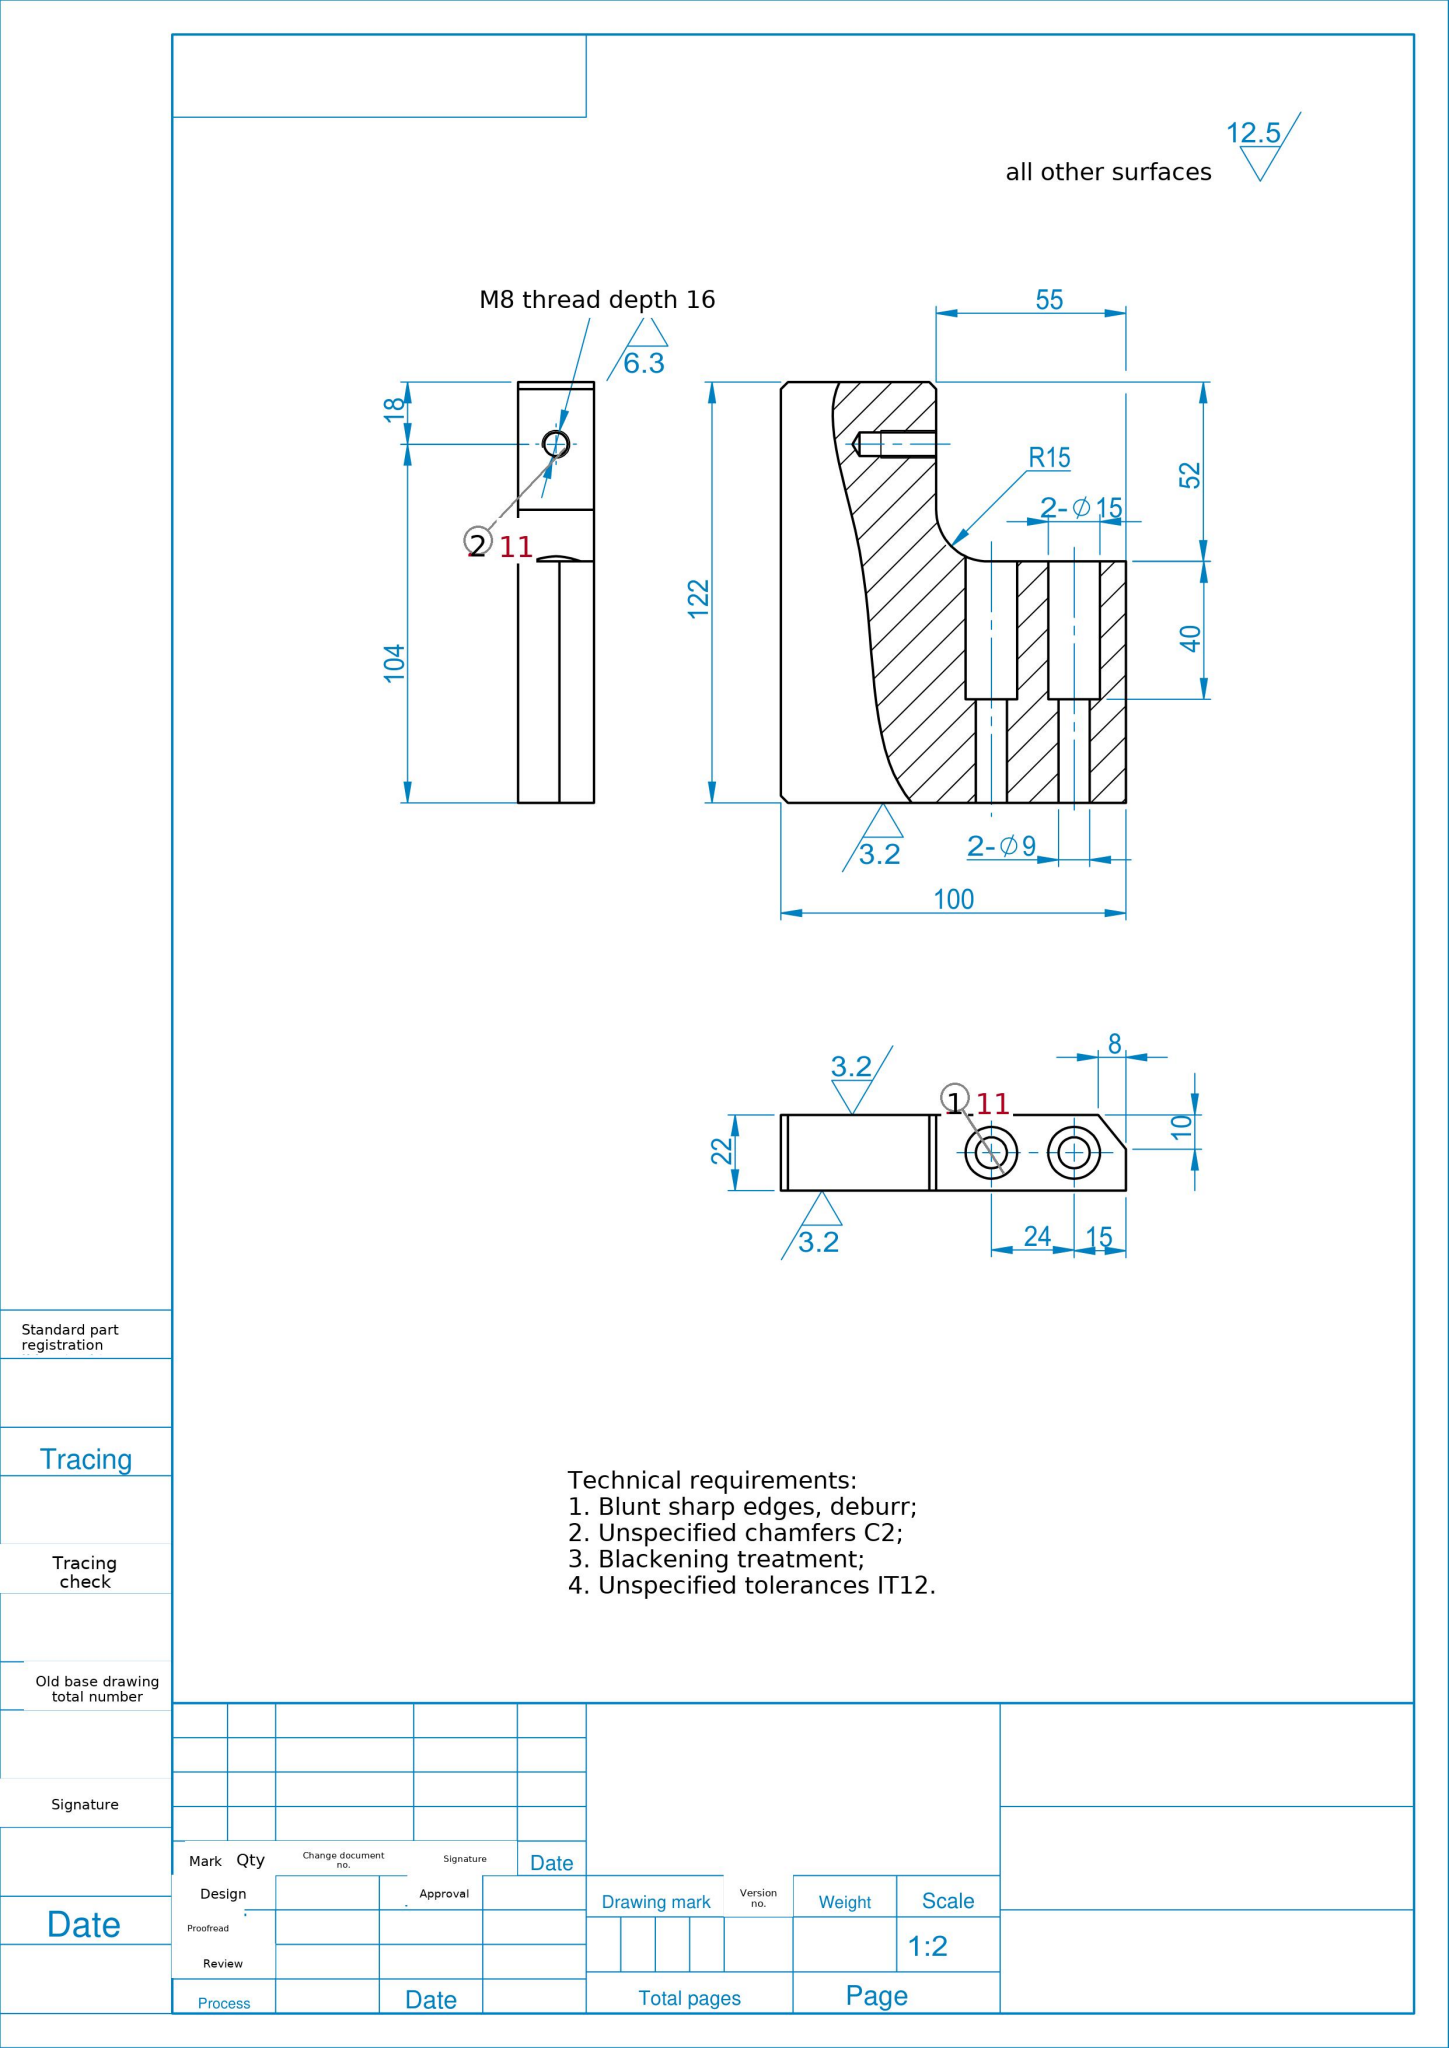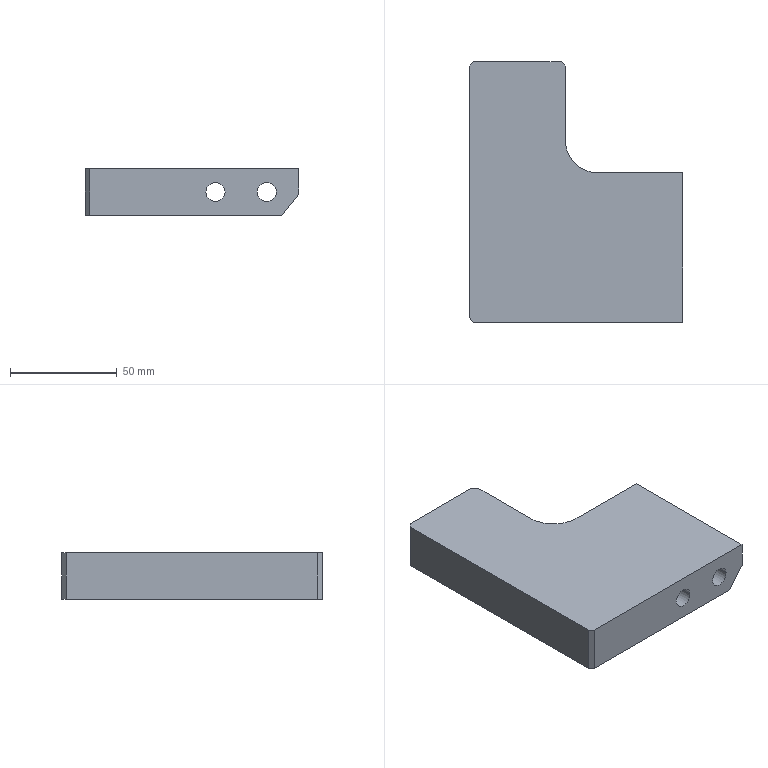Part | SolidWorks | mm | 1 solid | 27 faces | box 100 x 122 x 22 mm | volume 184797 mm3 | plane 14 | cylinder 11 | cone 2 | commonest cylinder face diameters 15 x4 9 x4 6.8 x2 30 x1
STEP:
#1=CARTESIAN_POINT('',(22.75,104.,14.4));
#2=VERTEX_POINT('',#1);
#3=CARTESIAN_POINT('',(22.75,104.,7.6));
#4=VERTEX_POINT('',#3);
#5=CARTESIAN_POINT('',(22.75,104.,11.));
#6=DIRECTION('',(1.,0.,0.));
#7=DIRECTION('',(0.,0.,-1.));
#8=AXIS2_PLACEMENT_3D('',#5,#6,#7);
#9=CIRCLE('',#8,3.4);
#10=EDGE_CURVE('',#2,#4,#9,.T.);
#11=ORIENTED_EDGE('',*,*,#10,.F.);
#12=CARTESIAN_POINT('',(45.,104.,14.4));
#13=VERTEX_POINT('',#12);
#14=CARTESIAN_POINT('',(45.,104.,14.4));
#15=DIRECTION('',(1.,0.,0.));
#16=VECTOR('',#15,1000.);
#17=LINE('',#14,#16);
#18=EDGE_CURVE('',#2,#13,#17,.T.);
#19=ORIENTED_EDGE('',*,*,#18,.T.);
#20=CARTESIAN_POINT('',(45.,104.,7.6));
#21=VERTEX_POINT('',#20);
#22=CARTESIAN_POINT('',(45.,104.,11.));
#23=DIRECTION('',(1.,0.,0.));
#24=DIRECTION('',(0.,0.,-1.));
#25=AXIS2_PLACEMENT_3D('',#22,#23,#24);
#26=CIRCLE('',#25,3.4);
#27=EDGE_CURVE('',#13,#21,#26,.T.);
#28=ORIENTED_EDGE('',*,*,#27,.T.);
#29=CARTESIAN_POINT('',(45.,104.,7.6));
#30=DIRECTION('',(1.,0.,0.));
#31=VECTOR('',#30,1000.);
#32=LINE('',#29,#31);
#33=EDGE_CURVE('',#4,#21,#32,.T.);
#34=ORIENTED_EDGE('',*,*,#33,.F.);
#35=EDGE_LOOP('',(#11,#19,#28,#34));
#36=FACE_OUTER_BOUND('',#35,.T.);
#37=CARTESIAN_POINT('',(45.,104.,11.));
#38=DIRECTION('',(1.,0.,0.));
#39=DIRECTION('',(0.,0.,-1.));
#40=AXIS2_PLACEMENT_3D('',#37,#38,#39);
#41=CYLINDRICAL_SURFACE('',#40,3.4);
#42=ADVANCED_FACE('',(#36),#41,.F.);
#43=CARTESIAN_POINT('',(20.707,104.,11.));
#44=VERTEX_POINT('',#43);
#45=CARTESIAN_POINT('',(22.75,104.,7.6));
#46=DIRECTION('',(0.515,0.,-0.8572));
#47=VECTOR('',#46,1000.);
#48=LINE('',#45,#47);
#49=EDGE_CURVE('',#44,#4,#48,.T.);
#50=ORIENTED_EDGE('',*,*,#49,.F.);
#51=CARTESIAN_POINT('',(22.75,104.,14.4));
#52=DIRECTION('',(0.515,0.,0.8572));
#53=VECTOR('',#52,1000.);
#54=LINE('',#51,#53);
#55=EDGE_CURVE('',#44,#2,#54,.T.);
#56=ORIENTED_EDGE('',*,*,#55,.T.);
#57=ORIENTED_EDGE('',*,*,#10,.T.);
#58=EDGE_LOOP('',(#50,#56,#57));
#59=FACE_OUTER_BOUND('',#58,.T.);
#60=CARTESIAN_POINT('',(22.75,104.,11.));
#61=DIRECTION('',(1.,0.,0.));
#62=DIRECTION('',(0.,0.,-1.));
#63=AXIS2_PLACEMENT_3D('',#60,#61,#62);
#64=CONICAL_SURFACE('',#63,3.4,1.03);
#65=ADVANCED_FACE('',(#59),#64,.F.);
#66=CARTESIAN_POINT('',(92.5,30.,11.));
#67=VERTEX_POINT('',#66);
#68=CARTESIAN_POINT('',(77.5,30.,11.));
#69=VERTEX_POINT('',#68);
#70=CARTESIAN_POINT('',(85.,30.,11.));
#71=DIRECTION('',(-0.,1.,0.));
#72=DIRECTION('',(-1.,-0.,0.));
#73=AXIS2_PLACEMENT_3D('',#70,#71,#72);
#74=CIRCLE('',#73,7.5);
#75=EDGE_CURVE('',#67,#69,#74,.T.);
#76=ORIENTED_EDGE('',*,*,#75,.F.);
#77=CARTESIAN_POINT('',(92.5,70.,11.));
#78=VERTEX_POINT('',#77);
#79=CARTESIAN_POINT('',(92.5,30.,11.));
#80=DIRECTION('',(-0.,1.,0.));
#81=VECTOR('',#80,1000.);
#82=LINE('',#79,#81);
#83=EDGE_CURVE('',#67,#78,#82,.T.);
#84=ORIENTED_EDGE('',*,*,#83,.T.);
#85=CARTESIAN_POINT('',(77.5,70.,11.));
#86=VERTEX_POINT('',#85);
#87=CARTESIAN_POINT('',(85.,70.,11.));
#88=DIRECTION('',(0.,-1.,0.));
#89=DIRECTION('',(1.,0.,0.));
#90=AXIS2_PLACEMENT_3D('',#87,#88,#89);
#91=CIRCLE('',#90,7.5);
#92=EDGE_CURVE('',#86,#78,#91,.T.);
#93=ORIENTED_EDGE('',*,*,#92,.F.);
#94=CARTESIAN_POINT('',(77.5,30.,11.));
#95=DIRECTION('',(-0.,1.,0.));
#96=VECTOR('',#95,1000.);
#97=LINE('',#94,#96);
#98=EDGE_CURVE('',#69,#86,#97,.T.);
#99=ORIENTED_EDGE('',*,*,#98,.F.);
#100=EDGE_LOOP('',(#76,#84,#93,#99));
#101=FACE_OUTER_BOUND('',#100,.T.);
#102=CARTESIAN_POINT('',(85.,30.,11.));
#103=DIRECTION('',(-0.,1.,0.));
#104=DIRECTION('',(-1.,-0.,0.));
#105=AXIS2_PLACEMENT_3D('',#102,#103,#104);
#106=CYLINDRICAL_SURFACE('',#105,7.5);
#107=ADVANCED_FACE('',(#101),#106,.F.);
#108=CARTESIAN_POINT('',(68.5,30.,11.));
#109=VERTEX_POINT('',#108);
#110=CARTESIAN_POINT('',(53.5,30.,11.));
#111=VERTEX_POINT('',#110);
#112=CARTESIAN_POINT('',(61.,30.,11.));
#113=DIRECTION('',(-0.,1.,0.));
#114=DIRECTION('',(-1.,-0.,0.));
#115=AXIS2_PLACEMENT_3D('',#112,#113,#114);
#116=CIRCLE('',#115,7.5);
#117=EDGE_CURVE('',#109,#111,#116,.T.);
#118=ORIENTED_EDGE('',*,*,#117,.F.);
#119=CARTESIAN_POINT('',(68.5,70.,11.));
#120=VERTEX_POINT('',#119);
#121=CARTESIAN_POINT('',(68.5,30.,11.));
#122=DIRECTION('',(-0.,1.,0.));
#123=VECTOR('',#122,1000.);
#124=LINE('',#121,#123);
#125=EDGE_CURVE('',#109,#120,#124,.T.);
#126=ORIENTED_EDGE('',*,*,#125,.T.);
#127=CARTESIAN_POINT('',(60.,70.,3.567));
#128=VERTEX_POINT('',#127);
#129=CARTESIAN_POINT('',(61.,70.,11.));
#130=DIRECTION('',(0.,-1.,0.));
#131=DIRECTION('',(1.,0.,0.));
#132=AXIS2_PLACEMENT_3D('',#129,#130,#131);
#133=CIRCLE('',#132,7.5);
#134=EDGE_CURVE('',#128,#120,#133,.T.);
#135=ORIENTED_EDGE('',*,*,#134,.F.);
#136=CARTESIAN_POINT('',(53.5,71.481,11.));
#137=VERTEX_POINT('',#136);
#138=CARTESIAN_POINT('',(53.5,71.481,11.));
#139=CARTESIAN_POINT('',(53.5,71.481,10.541));
#140=CARTESIAN_POINT('',(53.542,71.461,10.09));
#141=CARTESIAN_POINT('',(53.664,71.404,9.426));
#142=CARTESIAN_POINT('',(53.714,71.38,9.206));
#143=CARTESIAN_POINT('',(53.835,71.325,8.771));
#144=CARTESIAN_POINT('',(53.906,71.293,8.554));
#145=CARTESIAN_POINT('',(54.146,71.188,7.922));
#146=CARTESIAN_POINT('',(54.341,71.106,7.522));
#147=CARTESIAN_POINT('',(54.799,70.929,6.759));
#148=CARTESIAN_POINT('',(55.064,70.832,6.394));
#149=CARTESIAN_POINT('',(55.649,70.642,5.726));
#150=CARTESIAN_POINT('',(55.968,70.547,5.42));
#151=CARTESIAN_POINT('',(56.665,70.371,4.864));
#152=CARTESIAN_POINT('',(57.043,70.289,4.613));
#153=CARTESIAN_POINT('',(57.83,70.152,4.188));
#154=CARTESIAN_POINT('',(58.241,70.097,4.011));
#155=CARTESIAN_POINT('',(58.887,70.04,3.8));
#156=CARTESIAN_POINT('',(59.108,70.025,3.739));
#157=CARTESIAN_POINT('',(59.553,70.005,3.637));
#158=CARTESIAN_POINT('',(59.776,70.,3.597));
#159=CARTESIAN_POINT('',(60.,70.,3.567));
#160=B_SPLINE_CURVE_WITH_KNOTS('',3,(#138,#139,#140,#141,#142,#143,#144,#145,#146,#147,#148,#149,#150,#151,#152,#153,#154,#155,#156,#157,#158,#159),.UNSPECIFIED.,.F.,.F.,(4,2,2,2,2,2,2,2,2,2,4),(0.,0.001356,0.002034,0.002712,0.004067,0.005423,0.006779,0.008135,0.009491,0.01017,0.01085),.UNSPECIFIED.);
#161=EDGE_CURVE('',#137,#128,#160,.T.);
#162=ORIENTED_EDGE('',*,*,#161,.F.);
#163=CARTESIAN_POINT('',(53.5,30.,11.));
#164=DIRECTION('',(-0.,1.,0.));
#165=VECTOR('',#164,1000.);
#166=LINE('',#163,#165);
#167=EDGE_CURVE('',#111,#137,#166,.T.);
#168=ORIENTED_EDGE('',*,*,#167,.F.);
#169=EDGE_LOOP('',(#118,#126,#135,#162,#168));
#170=FACE_OUTER_BOUND('',#169,.T.);
#171=CARTESIAN_POINT('',(61.,30.,11.));
#172=DIRECTION('',(-0.,1.,0.));
#173=DIRECTION('',(-1.,-0.,0.));
#174=AXIS2_PLACEMENT_3D('',#171,#172,#173);
#175=CYLINDRICAL_SURFACE('',#174,7.5);
#176=ADVANCED_FACE('',(#170),#175,.F.);
#177=CARTESIAN_POINT('',(65.5,30.,11.));
#178=VERTEX_POINT('',#177);
#179=CARTESIAN_POINT('',(56.5,30.,11.));
#180=VERTEX_POINT('',#179);
#181=CARTESIAN_POINT('',(61.,30.,11.));
#182=DIRECTION('',(-0.,1.,0.));
#183=DIRECTION('',(-1.,0.,0.));
#184=AXIS2_PLACEMENT_3D('',#181,#182,#183);
#185=CIRCLE('',#184,4.5);
#186=EDGE_CURVE('',#178,#180,#185,.T.);
#187=ORIENTED_EDGE('',*,*,#186,.T.);
#188=CARTESIAN_POINT('',(56.5,-0.,11.));
#189=VERTEX_POINT('',#188);
#190=CARTESIAN_POINT('',(56.5,80.,11.));
#191=DIRECTION('',(0.,-1.,0.));
#192=VECTOR('',#191,1000.);
#193=LINE('',#190,#192);
#194=EDGE_CURVE('',#180,#189,#193,.T.);
#195=ORIENTED_EDGE('',*,*,#194,.T.);
#196=CARTESIAN_POINT('',(65.5,-0.,11.));
#197=VERTEX_POINT('',#196);
#198=CARTESIAN_POINT('',(61.,-0.,11.));
#199=DIRECTION('',(-0.,1.,0.));
#200=DIRECTION('',(-1.,-0.,0.));
#201=AXIS2_PLACEMENT_3D('',#198,#199,#200);
#202=CIRCLE('',#201,4.5);
#203=EDGE_CURVE('',#197,#189,#202,.T.);
#204=ORIENTED_EDGE('',*,*,#203,.F.);
#205=CARTESIAN_POINT('',(65.5,80.,11.));
#206=DIRECTION('',(0.,-1.,0.));
#207=VECTOR('',#206,1000.);
#208=LINE('',#205,#207);
#209=EDGE_CURVE('',#178,#197,#208,.T.);
#210=ORIENTED_EDGE('',*,*,#209,.F.);
#211=EDGE_LOOP('',(#187,#195,#204,#210));
#212=FACE_OUTER_BOUND('',#211,.T.);
#213=CARTESIAN_POINT('',(61.,80.,11.));
#214=DIRECTION('',(0.,-1.,0.));
#215=DIRECTION('',(1.,0.,0.));
#216=AXIS2_PLACEMENT_3D('',#213,#214,#215);
#217=CYLINDRICAL_SURFACE('',#216,4.5);
#218=ADVANCED_FACE('',(#212),#217,.F.);
#219=CARTESIAN_POINT('',(89.5,30.,11.));
#220=VERTEX_POINT('',#219);
#221=CARTESIAN_POINT('',(80.5,30.,11.));
#222=VERTEX_POINT('',#221);
#223=CARTESIAN_POINT('',(85.,30.,11.));
#224=DIRECTION('',(-0.,1.,0.));
#225=DIRECTION('',(-1.,0.,0.));
#226=AXIS2_PLACEMENT_3D('',#223,#224,#225);
#227=CIRCLE('',#226,4.5);
#228=EDGE_CURVE('',#220,#222,#227,.T.);
#229=ORIENTED_EDGE('',*,*,#228,.T.);
#230=CARTESIAN_POINT('',(80.5,-0.,11.));
#231=VERTEX_POINT('',#230);
#232=CARTESIAN_POINT('',(80.5,80.,11.));
#233=DIRECTION('',(0.,-1.,0.));
#234=VECTOR('',#233,1000.);
#235=LINE('',#232,#234);
#236=EDGE_CURVE('',#222,#231,#235,.T.);
#237=ORIENTED_EDGE('',*,*,#236,.T.);
#238=CARTESIAN_POINT('',(89.5,0.,11.));
#239=VERTEX_POINT('',#238);
#240=CARTESIAN_POINT('',(85.,0.,11.));
#241=DIRECTION('',(-0.,1.,0.));
#242=DIRECTION('',(-1.,-0.,0.));
#243=AXIS2_PLACEMENT_3D('',#240,#241,#242);
#244=CIRCLE('',#243,4.5);
#245=EDGE_CURVE('',#239,#231,#244,.T.);
#246=ORIENTED_EDGE('',*,*,#245,.F.);
#247=CARTESIAN_POINT('',(89.5,80.,11.));
#248=DIRECTION('',(0.,-1.,0.));
#249=VECTOR('',#248,1000.);
#250=LINE('',#247,#249);
#251=EDGE_CURVE('',#220,#239,#250,.T.);
#252=ORIENTED_EDGE('',*,*,#251,.F.);
#253=EDGE_LOOP('',(#229,#237,#246,#252));
#254=FACE_OUTER_BOUND('',#253,.T.);
#255=CARTESIAN_POINT('',(85.,80.,11.));
#256=DIRECTION('',(0.,-1.,0.));
#257=DIRECTION('',(1.,0.,0.));
#258=AXIS2_PLACEMENT_3D('',#255,#256,#257);
#259=CYLINDRICAL_SURFACE('',#258,4.5);
#260=ADVANCED_FACE('',(#254),#259,.F.);
#261=ORIENTED_EDGE('',*,*,#236,.F.);
#262=CARTESIAN_POINT('',(85.,30.,11.));
#263=DIRECTION('',(-0.,1.,0.));
#264=DIRECTION('',(-1.,0.,0.));
#265=AXIS2_PLACEMENT_3D('',#262,#263,#264);
#266=CIRCLE('',#265,4.5);
#267=EDGE_CURVE('',#222,#220,#266,.T.);
#268=ORIENTED_EDGE('',*,*,#267,.T.);
#269=ORIENTED_EDGE('',*,*,#251,.T.);
#270=CARTESIAN_POINT('',(85.,0.,11.));
#271=DIRECTION('',(-0.,1.,0.));
#272=DIRECTION('',(-1.,-0.,0.));
#273=AXIS2_PLACEMENT_3D('',#270,#271,#272);
#274=CIRCLE('',#273,4.5);
#275=EDGE_CURVE('',#231,#239,#274,.T.);
#276=ORIENTED_EDGE('',*,*,#275,.F.);
#277=EDGE_LOOP('',(#261,#268,#269,#276));
#278=FACE_OUTER_BOUND('',#277,.T.);
#279=CARTESIAN_POINT('',(85.,80.,11.));
#280=DIRECTION('',(0.,-1.,0.));
#281=DIRECTION('',(1.,0.,0.));
#282=AXIS2_PLACEMENT_3D('',#279,#280,#281);
#283=CYLINDRICAL_SURFACE('',#282,4.5);
#284=ADVANCED_FACE('',(#278),#283,.F.);
#285=ORIENTED_EDGE('',*,*,#194,.F.);
#286=CARTESIAN_POINT('',(61.,30.,11.));
#287=DIRECTION('',(-0.,1.,0.));
#288=DIRECTION('',(-1.,0.,0.));
#289=AXIS2_PLACEMENT_3D('',#286,#287,#288);
#290=CIRCLE('',#289,4.5);
#291=EDGE_CURVE('',#180,#178,#290,.T.);
#292=ORIENTED_EDGE('',*,*,#291,.T.);
#293=ORIENTED_EDGE('',*,*,#209,.T.);
#294=CARTESIAN_POINT('',(61.,-0.,11.));
#295=DIRECTION('',(-0.,1.,0.));
#296=DIRECTION('',(-1.,-0.,0.));
#297=AXIS2_PLACEMENT_3D('',#294,#295,#296);
#298=CIRCLE('',#297,4.5);
#299=EDGE_CURVE('',#189,#197,#298,.T.);
#300=ORIENTED_EDGE('',*,*,#299,.F.);
#301=EDGE_LOOP('',(#285,#292,#293,#300));
#302=FACE_OUTER_BOUND('',#301,.T.);
#303=CARTESIAN_POINT('',(61.,80.,11.));
#304=DIRECTION('',(0.,-1.,0.));
#305=DIRECTION('',(1.,0.,0.));
#306=AXIS2_PLACEMENT_3D('',#303,#304,#305);
#307=CYLINDRICAL_SURFACE('',#306,4.5);
#308=ADVANCED_FACE('',(#302),#307,.F.);
#309=ORIENTED_EDGE('',*,*,#203,.T.);
#310=ORIENTED_EDGE('',*,*,#299,.T.);
#311=EDGE_LOOP('',(#309,#310));
#312=FACE_BOUND('',#311,.T.);
#313=CARTESIAN_POINT('',(2.,0.,22.));
#314=VERTEX_POINT('',#313);
#315=CARTESIAN_POINT('',(100.,0.,22.));
#316=VERTEX_POINT('',#315);
#317=CARTESIAN_POINT('',(100.,0.,22.));
#318=DIRECTION('',(1.,0.,0.));
#319=VECTOR('',#318,1000.);
#320=LINE('',#317,#319);
#321=EDGE_CURVE('',#314,#316,#320,.T.);
#322=ORIENTED_EDGE('',*,*,#321,.F.);
#323=CARTESIAN_POINT('',(2.,0.,0.));
#324=VERTEX_POINT('',#323);
#325=CARTESIAN_POINT('',(2.,0.,22.));
#326=DIRECTION('',(0.,0.,-1.));
#327=VECTOR('',#326,1000.);
#328=LINE('',#325,#327);
#329=EDGE_CURVE('',#314,#324,#328,.T.);
#330=ORIENTED_EDGE('',*,*,#329,.T.);
#331=CARTESIAN_POINT('',(92.,0.,0.));
#332=VERTEX_POINT('',#331);
#333=CARTESIAN_POINT('',(100.,0.,0.));
#334=DIRECTION('',(1.,0.,0.));
#335=VECTOR('',#334,1000.);
#336=LINE('',#333,#335);
#337=EDGE_CURVE('',#324,#332,#336,.T.);
#338=ORIENTED_EDGE('',*,*,#337,.T.);
#339=CARTESIAN_POINT('',(100.,0.,10.));
#340=VERTEX_POINT('',#339);
#341=CARTESIAN_POINT('',(92.,0.,0.));
#342=DIRECTION('',(0.6247,0.,0.7809));
#343=VECTOR('',#342,1000.);
#344=LINE('',#341,#343);
#345=EDGE_CURVE('',#332,#340,#344,.T.);
#346=ORIENTED_EDGE('',*,*,#345,.T.);
#347=CARTESIAN_POINT('',(100.,0.,22.));
#348=DIRECTION('',(0.,0.,-1.));
#349=VECTOR('',#348,1000.);
#350=LINE('',#347,#349);
#351=EDGE_CURVE('',#316,#340,#350,.T.);
#352=ORIENTED_EDGE('',*,*,#351,.F.);
#353=EDGE_LOOP('',(#322,#330,#338,#346,#352));
#354=FACE_OUTER_BOUND('',#353,.T.);
#355=ORIENTED_EDGE('',*,*,#245,.T.);
#356=ORIENTED_EDGE('',*,*,#275,.T.);
#357=EDGE_LOOP('',(#355,#356));
#358=FACE_BOUND('',#357,.T.);
#359=CARTESIAN_POINT('',(100.,0.,22.));
#360=DIRECTION('',(-0.,1.,0.));
#361=DIRECTION('',(-1.,-0.,0.));
#362=AXIS2_PLACEMENT_3D('',#359,#360,#361);
#363=PLANE('',#362);
#364=ADVANCED_FACE('',(#312,#354,#358),#363,.F.);
#365=ORIENTED_EDGE('',*,*,#92,.T.);
#366=CARTESIAN_POINT('',(85.,70.,11.));
#367=DIRECTION('',(0.,-1.,0.));
#368=DIRECTION('',(1.,0.,0.));
#369=AXIS2_PLACEMENT_3D('',#366,#367,#368);
#370=CIRCLE('',#369,7.5);
#371=EDGE_CURVE('',#78,#86,#370,.T.);
#372=ORIENTED_EDGE('',*,*,#371,.T.);
#373=EDGE_LOOP('',(#365,#372));
#374=FACE_BOUND('',#373,.T.);
#375=CARTESIAN_POINT('',(60.,70.,0.));
#376=VERTEX_POINT('',#375);
#377=CARTESIAN_POINT('',(60.,70.,22.));
#378=DIRECTION('',(0.,0.,1.));
#379=VECTOR('',#378,1000.);
#380=LINE('',#377,#379);
#381=EDGE_CURVE('',#376,#128,#380,.T.);
#382=ORIENTED_EDGE('',*,*,#381,.T.);
#383=ORIENTED_EDGE('',*,*,#134,.T.);
#384=CARTESIAN_POINT('',(60.,70.,18.433));
#385=VERTEX_POINT('',#384);
#386=CARTESIAN_POINT('',(61.,70.,11.));
#387=DIRECTION('',(0.,-1.,0.));
#388=DIRECTION('',(1.,0.,0.));
#389=AXIS2_PLACEMENT_3D('',#386,#387,#388);
#390=CIRCLE('',#389,7.5);
#391=EDGE_CURVE('',#120,#385,#390,.T.);
#392=ORIENTED_EDGE('',*,*,#391,.T.);
#393=CARTESIAN_POINT('',(60.,70.,22.));
#394=VERTEX_POINT('',#393);
#395=CARTESIAN_POINT('',(60.,70.,22.));
#396=DIRECTION('',(0.,0.,1.));
#397=VECTOR('',#396,1000.);
#398=LINE('',#395,#397);
#399=EDGE_CURVE('',#385,#394,#398,.T.);
#400=ORIENTED_EDGE('',*,*,#399,.T.);
#401=CARTESIAN_POINT('',(100.,70.,22.));
#402=VERTEX_POINT('',#401);
#403=CARTESIAN_POINT('',(45.,70.,22.));
#404=DIRECTION('',(-1.,-0.,0.));
#405=VECTOR('',#404,1000.);
#406=LINE('',#403,#405);
#407=EDGE_CURVE('',#402,#394,#406,.T.);
#408=ORIENTED_EDGE('',*,*,#407,.F.);
#409=CARTESIAN_POINT('',(100.,70.,10.));
#410=VERTEX_POINT('',#409);
#411=CARTESIAN_POINT('',(100.,70.,22.));
#412=DIRECTION('',(0.,0.,-1.));
#413=VECTOR('',#412,1000.);
#414=LINE('',#411,#413);
#415=EDGE_CURVE('',#402,#410,#414,.T.);
#416=ORIENTED_EDGE('',*,*,#415,.T.);
#417=CARTESIAN_POINT('',(92.,70.,0.));
#418=VERTEX_POINT('',#417);
#419=CARTESIAN_POINT('',(92.,70.,0.));
#420=DIRECTION('',(0.6247,0.,0.7809));
#421=VECTOR('',#420,1000.);
#422=LINE('',#419,#421);
#423=EDGE_CURVE('',#418,#410,#422,.T.);
#424=ORIENTED_EDGE('',*,*,#423,.F.);
#425=CARTESIAN_POINT('',(45.,70.,0.));
#426=DIRECTION('',(-1.,-0.,0.));
#427=VECTOR('',#426,1000.);
#428=LINE('',#425,#427);
#429=EDGE_CURVE('',#418,#376,#428,.T.);
#430=ORIENTED_EDGE('',*,*,#429,.T.);
#431=EDGE_LOOP('',(#382,#383,#392,#400,#408,#416,#424,#430));
#432=FACE_OUTER_BOUND('',#431,.T.);
#433=CARTESIAN_POINT('',(45.,70.,22.));
#434=DIRECTION('',(0.,-1.,0.));
#435=DIRECTION('',(1.,0.,0.));
#436=AXIS2_PLACEMENT_3D('',#433,#434,#435);
#437=PLANE('',#436);
#438=ADVANCED_FACE('',(#374,#432),#437,.F.);
#439=ORIENTED_EDGE('',*,*,#399,.F.);
#440=CARTESIAN_POINT('',(60.,70.,18.433));
#441=CARTESIAN_POINT('',(59.547,70.,18.372));
#442=CARTESIAN_POINT('',(59.103,70.021,18.27));
#443=CARTESIAN_POINT('',(58.461,70.078,18.061));
#444=CARTESIAN_POINT('',(58.25,70.101,17.981));
#445=CARTESIAN_POINT('',(57.835,70.156,17.803));
#446=CARTESIAN_POINT('',(57.63,70.187,17.704));
#447=CARTESIAN_POINT('',(57.036,70.29,17.383));
#448=CARTESIAN_POINT('',(56.665,70.371,17.136));
#449=CARTESIAN_POINT('',(55.969,70.547,16.58));
#450=CARTESIAN_POINT('',(55.644,70.643,16.269));
#451=CARTESIAN_POINT('',(55.061,70.833,15.602));
#452=CARTESIAN_POINT('',(54.801,70.928,15.245));
#453=CARTESIAN_POINT('',(54.456,71.061,14.672));
#454=CARTESIAN_POINT('',(54.349,71.105,14.473));
#455=CARTESIAN_POINT('',(54.153,71.186,14.07));
#456=CARTESIAN_POINT('',(54.065,71.224,13.865));
#457=CARTESIAN_POINT('',(53.828,71.327,13.239));
#458=CARTESIAN_POINT('',(53.707,71.383,12.808));
#459=CARTESIAN_POINT('',(53.543,71.461,11.917));
#460=CARTESIAN_POINT('',(53.5,71.481,11.457));
#461=CARTESIAN_POINT('',(53.5,71.481,11.));
#462=B_SPLINE_CURVE_WITH_KNOTS('',3,(#440,#441,#442,#443,#444,#445,#446,#447,#448,#449,#450,#451,#452,#453,#454,#455,#456,#457,#458,#459,#460,#461),.UNSPECIFIED.,.F.,.F.,(4,2,2,2,2,2,2,2,2,2,4),(0.03693,0.03828,0.03895,0.03963,0.04098,0.04233,0.04368,0.04436,0.04503,0.04638,0.04774),.UNSPECIFIED.);
#463=EDGE_CURVE('',#385,#137,#462,.T.);
#464=ORIENTED_EDGE('',*,*,#463,.T.);
#465=ORIENTED_EDGE('',*,*,#161,.T.);
#466=ORIENTED_EDGE('',*,*,#381,.F.);
#467=CARTESIAN_POINT('',(45.,85.,0.));
#468=VERTEX_POINT('',#467);
#469=CARTESIAN_POINT('',(60.,85.,0.));
#470=DIRECTION('',(0.,0.,1.));
#471=DIRECTION('',(-1.,0.,0.));
#472=AXIS2_PLACEMENT_3D('',#469,#470,#471);
#473=CIRCLE('',#472,15.);
#474=EDGE_CURVE('',#468,#376,#473,.T.);
#475=ORIENTED_EDGE('',*,*,#474,.F.);
#476=CARTESIAN_POINT('',(45.,85.,22.));
#477=VERTEX_POINT('',#476);
#478=CARTESIAN_POINT('',(45.,85.,0.));
#479=DIRECTION('',(0.,0.,-1.));
#480=VECTOR('',#479,1000.);
#481=LINE('',#478,#480);
#482=EDGE_CURVE('',#477,#468,#481,.T.);
#483=ORIENTED_EDGE('',*,*,#482,.F.);
#484=CARTESIAN_POINT('',(60.,85.,22.));
#485=DIRECTION('',(0.,0.,-1.));
#486=DIRECTION('',(-1.,0.,0.));
#487=AXIS2_PLACEMENT_3D('',#484,#485,#486);
#488=CIRCLE('',#487,15.);
#489=EDGE_CURVE('',#394,#477,#488,.T.);
#490=ORIENTED_EDGE('',*,*,#489,.F.);
#491=EDGE_LOOP('',(#439,#464,#465,#466,#475,#483,#490));
#492=FACE_OUTER_BOUND('',#491,.T.);
#493=CARTESIAN_POINT('',(60.,85.,22.));
#494=DIRECTION('',(0.,0.,1.));
#495=DIRECTION('',(1.,0.,0.));
#496=AXIS2_PLACEMENT_3D('',#493,#494,#495);
#497=CYLINDRICAL_SURFACE('',#496,15.);
#498=ADVANCED_FACE('',(#492),#497,.F.);
#499=CARTESIAN_POINT('',(0.,120.,22.));
#500=VERTEX_POINT('',#499);
#501=CARTESIAN_POINT('',(0.,2.,22.));
#502=VERTEX_POINT('',#501);
#503=CARTESIAN_POINT('',(0.,122.,22.));
#504=DIRECTION('',(0.,-1.,0.));
#505=VECTOR('',#504,1000.);
#506=LINE('',#503,#505);
#507=EDGE_CURVE('',#500,#502,#506,.T.);
#508=ORIENTED_EDGE('',*,*,#507,.F.);
#509=CARTESIAN_POINT('',(0.,120.,0.));
#510=VERTEX_POINT('',#509);
#511=CARTESIAN_POINT('',(0.,120.,22.));
#512=DIRECTION('',(0.,0.,-1.));
#513=VECTOR('',#512,1000.);
#514=LINE('',#511,#513);
#515=EDGE_CURVE('',#500,#510,#514,.T.);
#516=ORIENTED_EDGE('',*,*,#515,.T.);
#517=CARTESIAN_POINT('',(0.,2.,0.));
#518=VERTEX_POINT('',#517);
#519=CARTESIAN_POINT('',(0.,122.,0.));
#520=DIRECTION('',(0.,-1.,0.));
#521=VECTOR('',#520,1000.);
#522=LINE('',#519,#521);
#523=EDGE_CURVE('',#510,#518,#522,.T.);
#524=ORIENTED_EDGE('',*,*,#523,.T.);
#525=CARTESIAN_POINT('',(0.,2.,22.));
#526=DIRECTION('',(0.,0.,1.));
#527=VECTOR('',#526,1000.);
#528=LINE('',#525,#527);
#529=EDGE_CURVE('',#518,#502,#528,.T.);
#530=ORIENTED_EDGE('',*,*,#529,.T.);
#531=EDGE_LOOP('',(#508,#516,#524,#530));
#532=FACE_OUTER_BOUND('',#531,.T.);
#533=CARTESIAN_POINT('',(0.,122.,22.));
#534=DIRECTION('',(1.,0.,0.));
#535=DIRECTION('',(-0.,1.,0.));
#536=AXIS2_PLACEMENT_3D('',#533,#534,#535);
#537=PLANE('',#536);
#538=ADVANCED_FACE('',(#532),#537,.F.);
#539=ORIENTED_EDGE('',*,*,#351,.T.);
#540=CARTESIAN_POINT('',(100.,0.,10.));
#541=DIRECTION('',(-0.,1.,0.));
#542=VECTOR('',#541,1000.);
#543=LINE('',#540,#542);
#544=EDGE_CURVE('',#340,#410,#543,.T.);
#545=ORIENTED_EDGE('',*,*,#544,.T.);
#546=ORIENTED_EDGE('',*,*,#415,.F.);
#547=CARTESIAN_POINT('',(100.,70.,22.));
#548=DIRECTION('',(-0.,1.,0.));
#549=VECTOR('',#548,1000.);
#550=LINE('',#547,#549);
#551=EDGE_CURVE('',#316,#402,#550,.T.);
#552=ORIENTED_EDGE('',*,*,#551,.F.);
#553=EDGE_LOOP('',(#539,#545,#546,#552));
#554=FACE_OUTER_BOUND('',#553,.T.);
#555=CARTESIAN_POINT('',(100.,70.,22.));
#556=DIRECTION('',(-1.,-0.,0.));
#557=DIRECTION('',(0.,-1.,0.));
#558=AXIS2_PLACEMENT_3D('',#555,#556,#557);
#559=PLANE('',#558);
#560=ADVANCED_FACE('',(#554),#559,.F.);
#561=CARTESIAN_POINT('',(45.,104.,11.));
#562=DIRECTION('',(1.,0.,0.));
#563=DIRECTION('',(0.,0.,-1.));
#564=AXIS2_PLACEMENT_3D('',#561,#562,#563);
#565=CIRCLE('',#564,3.4);
#566=EDGE_CURVE('',#21,#13,#565,.T.);
#567=ORIENTED_EDGE('',*,*,#566,.F.);
#568=ORIENTED_EDGE('',*,*,#27,.F.);
#569=EDGE_LOOP('',(#567,#568));
#570=FACE_BOUND('',#569,.T.);
#571=CARTESIAN_POINT('',(45.,120.,22.));
#572=VERTEX_POINT('',#571);
#573=CARTESIAN_POINT('',(45.,122.,22.));
#574=DIRECTION('',(-0.,1.,0.));
#575=VECTOR('',#574,1000.);
#576=LINE('',#573,#575);
#577=EDGE_CURVE('',#477,#572,#576,.T.);
#578=ORIENTED_EDGE('',*,*,#577,.F.);
#579=ORIENTED_EDGE('',*,*,#482,.T.);
#580=CARTESIAN_POINT('',(45.,120.,0.));
#581=VERTEX_POINT('',#580);
#582=CARTESIAN_POINT('',(45.,122.,0.));
#583=DIRECTION('',(-0.,1.,0.));
#584=VECTOR('',#583,1000.);
#585=LINE('',#582,#584);
#586=EDGE_CURVE('',#468,#581,#585,.T.);
#587=ORIENTED_EDGE('',*,*,#586,.T.);
#588=CARTESIAN_POINT('',(45.,120.,22.));
#589=DIRECTION('',(0.,0.,1.));
#590=VECTOR('',#589,1000.);
#591=LINE('',#588,#590);
#592=EDGE_CURVE('',#581,#572,#591,.T.);
#593=ORIENTED_EDGE('',*,*,#592,.T.);
#594=EDGE_LOOP('',(#578,#579,#587,#593));
#595=FACE_OUTER_BOUND('',#594,.T.);
#596=CARTESIAN_POINT('',(45.,122.,22.));
#597=DIRECTION('',(-1.,-0.,0.));
#598=DIRECTION('',(0.,-1.,0.));
#599=AXIS2_PLACEMENT_3D('',#596,#597,#598);
#600=PLANE('',#599);
#601=ADVANCED_FACE('',(#570,#595),#600,.F.);
#602=CARTESIAN_POINT('',(43.,122.,22.));
#603=VERTEX_POINT('',#602);
#604=CARTESIAN_POINT('',(2.,122.,22.));
#605=VERTEX_POINT('',#604);
#606=CARTESIAN_POINT('',(0.,122.,22.));
#607=DIRECTION('',(-1.,0.,0.));
#608=VECTOR('',#607,1000.);
#609=LINE('',#606,#608);
#610=EDGE_CURVE('',#603,#605,#609,.T.);
#611=ORIENTED_EDGE('',*,*,#610,.F.);
#612=CARTESIAN_POINT('',(43.,122.,0.));
#613=VERTEX_POINT('',#612);
#614=CARTESIAN_POINT('',(43.,122.,22.));
#615=DIRECTION('',(0.,0.,-1.));
#616=VECTOR('',#615,1000.);
#617=LINE('',#614,#616);
#618=EDGE_CURVE('',#603,#613,#617,.T.);
#619=ORIENTED_EDGE('',*,*,#618,.T.);
#620=CARTESIAN_POINT('',(2.,122.,0.));
#621=VERTEX_POINT('',#620);
#622=CARTESIAN_POINT('',(0.,122.,0.));
#623=DIRECTION('',(-1.,0.,0.));
#624=VECTOR('',#623,1000.);
#625=LINE('',#622,#624);
#626=EDGE_CURVE('',#613,#621,#625,.T.);
#627=ORIENTED_EDGE('',*,*,#626,.T.);
#628=CARTESIAN_POINT('',(2.,122.,22.));
#629=DIRECTION('',(0.,0.,1.));
#630=VECTOR('',#629,1000.);
#631=LINE('',#628,#630);
#632=EDGE_CURVE('',#621,#605,#631,.T.);
#633=ORIENTED_EDGE('',*,*,#632,.T.);
#634=EDGE_LOOP('',(#611,#619,#627,#633));
#635=FACE_OUTER_BOUND('',#634,.T.);
#636=CARTESIAN_POINT('',(0.,122.,22.));
#637=DIRECTION('',(-0.,-1.,0.));
#638=DIRECTION('',(1.,-0.,0.));
#639=AXIS2_PLACEMENT_3D('',#636,#637,#638);
#640=PLANE('',#639);
#641=ADVANCED_FACE('',(#635),#640,.F.);
#642=ORIENTED_EDGE('',*,*,#407,.T.);
#643=ORIENTED_EDGE('',*,*,#489,.T.);
#644=ORIENTED_EDGE('',*,*,#577,.T.);
#645=CARTESIAN_POINT('',(43.,122.,22.));
#646=DIRECTION('',(-0.7071,0.7071,0.));
#647=VECTOR('',#646,1000.);
#648=LINE('',#645,#647);
#649=EDGE_CURVE('',#572,#603,#648,.T.);
#650=ORIENTED_EDGE('',*,*,#649,.T.);
#651=ORIENTED_EDGE('',*,*,#610,.T.);
#652=CARTESIAN_POINT('',(0.,120.,22.));
#653=DIRECTION('',(-0.7071,-0.7071,0.));
#654=VECTOR('',#653,1000.);
#655=LINE('',#652,#654);
#656=EDGE_CURVE('',#605,#500,#655,.T.);
#657=ORIENTED_EDGE('',*,*,#656,.T.);
#658=ORIENTED_EDGE('',*,*,#507,.T.);
#659=CARTESIAN_POINT('',(2.,0.,22.));
#660=DIRECTION('',(0.7071,-0.7071,0.));
#661=VECTOR('',#660,1000.);
#662=LINE('',#659,#661);
#663=EDGE_CURVE('',#502,#314,#662,.T.);
#664=ORIENTED_EDGE('',*,*,#663,.T.);
#665=ORIENTED_EDGE('',*,*,#321,.T.);
#666=ORIENTED_EDGE('',*,*,#551,.T.);
#667=EDGE_LOOP('',(#642,#643,#644,#650,#651,#657,#658,#664,#665,#666));
#668=FACE_OUTER_BOUND('',#667,.T.);
#669=CARTESIAN_POINT('',(0.,0.,22.));
#670=DIRECTION('',(0.,0.,-1.));
#671=DIRECTION('',(-1.,-0.,0.));
#672=AXIS2_PLACEMENT_3D('',#669,#670,#671);
#673=PLANE('',#672);
#674=ADVANCED_FACE('',(#668),#673,.F.);
#675=ORIENTED_EDGE('',*,*,#626,.F.);
#676=CARTESIAN_POINT('',(82.5,82.5,0.));
#677=DIRECTION('',(0.7071,-0.7071,0.));
#678=VECTOR('',#677,1000.);
#679=LINE('',#676,#678);
#680=EDGE_CURVE('',#613,#581,#679,.T.);
#681=ORIENTED_EDGE('',*,*,#680,.T.);
#682=ORIENTED_EDGE('',*,*,#586,.F.);
#683=ORIENTED_EDGE('',*,*,#474,.T.);
#684=ORIENTED_EDGE('',*,*,#429,.F.);
#685=CARTESIAN_POINT('',(92.,0.,0.));
#686=DIRECTION('',(-0.,1.,0.));
#687=VECTOR('',#686,1000.);
#688=LINE('',#685,#687);
#689=EDGE_CURVE('',#332,#418,#688,.T.);
#690=ORIENTED_EDGE('',*,*,#689,.F.);
#691=ORIENTED_EDGE('',*,*,#337,.F.);
#692=CARTESIAN_POINT('',(1.,1.,0.));
#693=DIRECTION('',(-0.7071,0.7071,0.));
#694=VECTOR('',#693,1000.);
#695=LINE('',#692,#694);
#696=EDGE_CURVE('',#324,#518,#695,.T.);
#697=ORIENTED_EDGE('',*,*,#696,.T.);
#698=ORIENTED_EDGE('',*,*,#523,.F.);
#699=CARTESIAN_POINT('',(-60.,60.,0.));
#700=DIRECTION('',(0.7071,0.7071,0.));
#701=VECTOR('',#700,1000.);
#702=LINE('',#699,#701);
#703=EDGE_CURVE('',#510,#621,#702,.T.);
#704=ORIENTED_EDGE('',*,*,#703,.T.);
#705=EDGE_LOOP('',(#675,#681,#682,#683,#684,#690,#691,#697,#698,#704));
#706=FACE_OUTER_BOUND('',#705,.T.);
#707=CARTESIAN_POINT('',(0.,0.,0.));
#708=DIRECTION('',(0.,0.,-1.));
#709=DIRECTION('',(-1.,-0.,0.));
#710=AXIS2_PLACEMENT_3D('',#707,#708,#709);
#711=PLANE('',#710);
#712=ADVANCED_FACE('',(#706),#711,.T.);
#713=ORIENTED_EDGE('',*,*,#423,.T.);
#714=ORIENTED_EDGE('',*,*,#544,.F.);
#715=ORIENTED_EDGE('',*,*,#345,.F.);
#716=ORIENTED_EDGE('',*,*,#689,.T.);
#717=EDGE_LOOP('',(#713,#714,#715,#716));
#718=FACE_OUTER_BOUND('',#717,.T.);
#719=CARTESIAN_POINT('',(92.,0.,0.));
#720=DIRECTION('',(-0.7809,-0.,0.6247));
#721=DIRECTION('',(0.6247,0.,0.7809));
#722=AXIS2_PLACEMENT_3D('',#719,#720,#721);
#723=PLANE('',#722);
#724=ADVANCED_FACE('',(#718),#723,.F.);
#725=ORIENTED_EDGE('',*,*,#663,.F.);
#726=ORIENTED_EDGE('',*,*,#529,.F.);
#727=ORIENTED_EDGE('',*,*,#696,.F.);
#728=ORIENTED_EDGE('',*,*,#329,.F.);
#729=EDGE_LOOP('',(#725,#726,#727,#728));
#730=FACE_OUTER_BOUND('',#729,.T.);
#731=CARTESIAN_POINT('',(2.,0.,22.));
#732=DIRECTION('',(0.7071,0.7071,0.));
#733=DIRECTION('',(0.,0.,-1.));
#734=AXIS2_PLACEMENT_3D('',#731,#732,#733);
#735=PLANE('',#734);
#736=ADVANCED_FACE('',(#730),#735,.F.);
#737=ORIENTED_EDGE('',*,*,#649,.F.);
#738=ORIENTED_EDGE('',*,*,#592,.F.);
#739=ORIENTED_EDGE('',*,*,#680,.F.);
#740=ORIENTED_EDGE('',*,*,#618,.F.);
#741=EDGE_LOOP('',(#737,#738,#739,#740));
#742=FACE_OUTER_BOUND('',#741,.T.);
#743=CARTESIAN_POINT('',(43.,122.,22.));
#744=DIRECTION('',(-0.7071,-0.7071,0.));
#745=DIRECTION('',(0.,0.,-1.));
#746=AXIS2_PLACEMENT_3D('',#743,#744,#745);
#747=PLANE('',#746);
#748=ADVANCED_FACE('',(#742),#747,.F.);
#749=ORIENTED_EDGE('',*,*,#656,.F.);
#750=ORIENTED_EDGE('',*,*,#632,.F.);
#751=ORIENTED_EDGE('',*,*,#703,.F.);
#752=ORIENTED_EDGE('',*,*,#515,.F.);
#753=EDGE_LOOP('',(#749,#750,#751,#752));
#754=FACE_OUTER_BOUND('',#753,.T.);
#755=CARTESIAN_POINT('',(0.,120.,22.));
#756=DIRECTION('',(0.7071,-0.7071,0.));
#757=DIRECTION('',(0.,0.,-1.));
#758=AXIS2_PLACEMENT_3D('',#755,#756,#757);
#759=PLANE('',#758);
#760=ADVANCED_FACE('',(#754),#759,.F.);
#761=ORIENTED_EDGE('',*,*,#125,.F.);
#762=CARTESIAN_POINT('',(61.,30.,11.));
#763=DIRECTION('',(-0.,1.,0.));
#764=DIRECTION('',(-1.,-0.,0.));
#765=AXIS2_PLACEMENT_3D('',#762,#763,#764);
#766=CIRCLE('',#765,7.5);
#767=EDGE_CURVE('',#111,#109,#766,.T.);
#768=ORIENTED_EDGE('',*,*,#767,.F.);
#769=ORIENTED_EDGE('',*,*,#167,.T.);
#770=ORIENTED_EDGE('',*,*,#463,.F.);
#771=ORIENTED_EDGE('',*,*,#391,.F.);
#772=EDGE_LOOP('',(#761,#768,#769,#770,#771));
#773=FACE_OUTER_BOUND('',#772,.T.);
#774=CARTESIAN_POINT('',(61.,30.,11.));
#775=DIRECTION('',(-0.,1.,0.));
#776=DIRECTION('',(-1.,-0.,0.));
#777=AXIS2_PLACEMENT_3D('',#774,#775,#776);
#778=CYLINDRICAL_SURFACE('',#777,7.5);
#779=ADVANCED_FACE('',(#773),#778,.F.);
#780=ORIENTED_EDGE('',*,*,#186,.F.);
#781=ORIENTED_EDGE('',*,*,#291,.F.);
#782=EDGE_LOOP('',(#780,#781));
#783=FACE_BOUND('',#782,.T.);
#784=ORIENTED_EDGE('',*,*,#767,.T.);
#785=ORIENTED_EDGE('',*,*,#117,.T.);
#786=EDGE_LOOP('',(#784,#785));
#787=FACE_OUTER_BOUND('',#786,.T.);
#788=CARTESIAN_POINT('',(61.,30.,11.));
#789=DIRECTION('',(-0.,1.,0.));
#790=DIRECTION('',(-1.,-0.,0.));
#791=AXIS2_PLACEMENT_3D('',#788,#789,#790);
#792=PLANE('',#791);
#793=ADVANCED_FACE('',(#783,#787),#792,.T.);
#794=ORIENTED_EDGE('',*,*,#83,.F.);
#795=CARTESIAN_POINT('',(85.,30.,11.));
#796=DIRECTION('',(-0.,1.,0.));
#797=DIRECTION('',(-1.,-0.,0.));
#798=AXIS2_PLACEMENT_3D('',#795,#796,#797);
#799=CIRCLE('',#798,7.5);
#800=EDGE_CURVE('',#69,#67,#799,.T.);
#801=ORIENTED_EDGE('',*,*,#800,.F.);
#802=ORIENTED_EDGE('',*,*,#98,.T.);
#803=ORIENTED_EDGE('',*,*,#371,.F.);
#804=EDGE_LOOP('',(#794,#801,#802,#803));
#805=FACE_OUTER_BOUND('',#804,.T.);
#806=CARTESIAN_POINT('',(85.,30.,11.));
#807=DIRECTION('',(-0.,1.,0.));
#808=DIRECTION('',(-1.,-0.,0.));
#809=AXIS2_PLACEMENT_3D('',#806,#807,#808);
#810=CYLINDRICAL_SURFACE('',#809,7.5);
#811=ADVANCED_FACE('',(#805),#810,.F.);
#812=ORIENTED_EDGE('',*,*,#228,.F.);
#813=ORIENTED_EDGE('',*,*,#267,.F.);
#814=EDGE_LOOP('',(#812,#813));
#815=FACE_BOUND('',#814,.T.);
#816=ORIENTED_EDGE('',*,*,#800,.T.);
#817=ORIENTED_EDGE('',*,*,#75,.T.);
#818=EDGE_LOOP('',(#816,#817));
#819=FACE_OUTER_BOUND('',#818,.T.);
#820=CARTESIAN_POINT('',(85.,30.,11.));
#821=DIRECTION('',(-0.,1.,0.));
#822=DIRECTION('',(-1.,-0.,0.));
#823=AXIS2_PLACEMENT_3D('',#820,#821,#822);
#824=PLANE('',#823);
#825=ADVANCED_FACE('',(#815,#819),#824,.T.);
#826=ORIENTED_EDGE('',*,*,#55,.F.);
#827=ORIENTED_EDGE('',*,*,#49,.T.);
#828=CARTESIAN_POINT('',(22.75,104.,11.));
#829=DIRECTION('',(1.,0.,0.));
#830=DIRECTION('',(0.,0.,-1.));
#831=AXIS2_PLACEMENT_3D('',#828,#829,#830);
#832=CIRCLE('',#831,3.4);
#833=EDGE_CURVE('',#4,#2,#832,.T.);
#834=ORIENTED_EDGE('',*,*,#833,.T.);
#835=EDGE_LOOP('',(#826,#827,#834));
#836=FACE_OUTER_BOUND('',#835,.T.);
#837=CARTESIAN_POINT('',(22.75,104.,11.));
#838=DIRECTION('',(1.,0.,0.));
#839=DIRECTION('',(0.,0.,-1.));
#840=AXIS2_PLACEMENT_3D('',#837,#838,#839);
#841=CONICAL_SURFACE('',#840,3.4,1.03);
#842=ADVANCED_FACE('',(#836),#841,.F.);
#843=ORIENTED_EDGE('',*,*,#18,.F.);
#844=ORIENTED_EDGE('',*,*,#833,.F.);
#845=ORIENTED_EDGE('',*,*,#33,.T.);
#846=ORIENTED_EDGE('',*,*,#566,.T.);
#847=EDGE_LOOP('',(#843,#844,#845,#846));
#848=FACE_OUTER_BOUND('',#847,.T.);
#849=CARTESIAN_POINT('',(45.,104.,11.));
#850=DIRECTION('',(1.,0.,0.));
#851=DIRECTION('',(0.,0.,-1.));
#852=AXIS2_PLACEMENT_3D('',#849,#850,#851);
#853=CYLINDRICAL_SURFACE('',#852,3.4);
#854=ADVANCED_FACE('',(#848),#853,.F.);
#855=CLOSED_SHELL('',(#42,#65,#107,#176,#218,#260,#284,#308,#364,#438,#498,#538,#560,#601,#641,#674,#712,#724,#736,#748,#760,#779,#793,#811,#825,#842,#854));
#856=MANIFOLD_SOLID_BREP('',#855);
#857=CARTESIAN_POINT('',(0.,0.,0.));
#858=DIRECTION('',(0.,0.,1.));
#859=DIRECTION('',(1.,0.,0.));
#860=AXIS2_PLACEMENT_3D('',#857,#858,#859);
#861=(LENGTH_UNIT()NAMED_UNIT(*)SI_UNIT(.MILLI.,.METRE.));
#862=UNCERTAINTY_MEASURE_WITH_UNIT(LENGTH_MEASURE(0.00001),#861,'','');
#863=(NAMED_UNIT(*)PLANE_ANGLE_UNIT()SI_UNIT($,.RADIAN.));
#864=(NAMED_UNIT(*)SI_UNIT($,.STERADIAN.)SOLID_ANGLE_UNIT());
#865=(GEOMETRIC_REPRESENTATION_CONTEXT(3)GLOBAL_UNCERTAINTY_ASSIGNED_CONTEXT((#862))GLOBAL_UNIT_ASSIGNED_CONTEXT((#861,#863,#864))REPRESENTATION_CONTEXT('',''));
#866=ADVANCED_BREP_SHAPE_REPRESENTATION('',(#856,#860),#865);